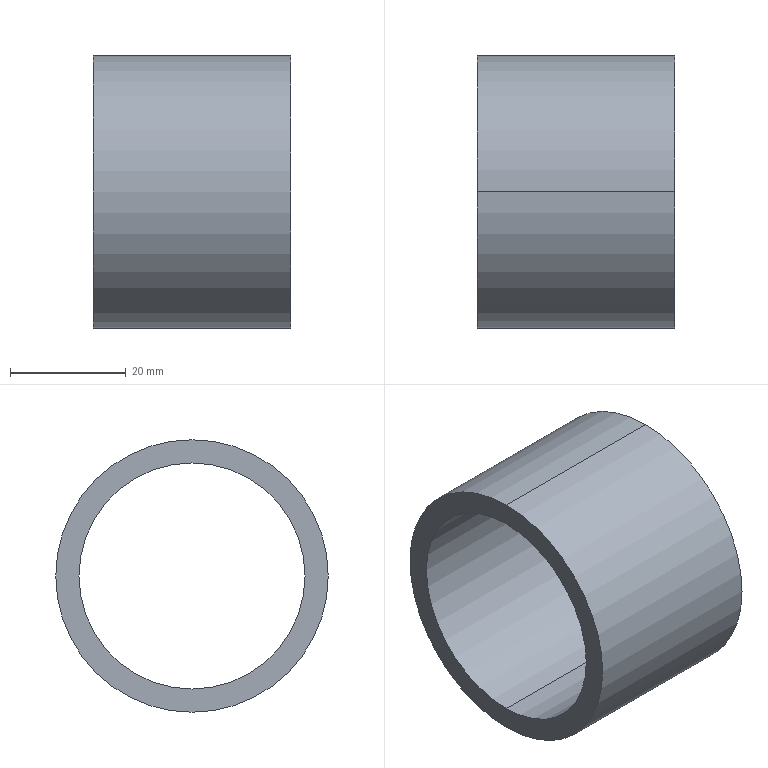Component | SolidWorks | 4-12-12ClampingAxisAssembly-1_4-12-6ClampingAxisBearingOuterPad-1 | 1 solid | 6 faces | box 34 x 47 x 47 mm | volume 18372 mm3 | cylinder 4 | plane 2 | commonest cylinder face diameters 39 x2 47 x2
build123d program:
from build123d import *

# Parameters (mm, degrees)
SKETCH1_R      = 23.5
SKETCH1_R_2    = 19.5
EXTRUDE1_DEPTH = 34


with BuildPart() as part:
    # Sketch1 → Extrude1 (new body)
    with BuildSketch(Plane(origin=(0, 0, 0), x_dir=(1, 0, 0), z_dir=(0, 1, 0))):
        with Locations(Location((0, 0, 0), (0, 0, 270))):
            Circle(SKETCH1_R)
        with Locations(Location((0, 0, 0), (0, 0, 270))):
            Circle(SKETCH1_R_2, mode=Mode.SUBTRACT)
    extrude(amount=EXTRUDE1_DEPTH)


solid = part.part

# Placed as in the assembly
solid = solid.moved(Location((-67.809, -4.181, 0), (0, 0, 90)))
STEP:
#1=COLOUR_RGB('',0.7922,0.8196,0.9333);
#2=FILL_AREA_STYLE_COLOUR('',#1);
#3=FILL_AREA_STYLE('',(#2));
#4=SURFACE_STYLE_FILL_AREA(#3);
#5=SURFACE_SIDE_STYLE('',(#4));
#6=SURFACE_STYLE_USAGE(.BOTH.,#5);
#7=PRESENTATION_STYLE_ASSIGNMENT((#6));
#8=CARTESIAN_POINT('',(-4.008,-0.1646,-0.7677));
#9=VERTEX_POINT('',#8);
#10=CARTESIAN_POINT('',(-4.008,-0.1646,0.7677));
#11=VERTEX_POINT('',#10);
#12=CARTESIAN_POINT('',(-4.008,-0.1646,0.));
#13=DIRECTION('',(-1.,-0.,-0.));
#14=DIRECTION('',(0.,0.,1.));
#15=AXIS2_PLACEMENT_3D('',#12,#13,#14);
#16=CIRCLE('',#15,0.7677);
#17=EDGE_CURVE('',#9,#11,#16,.T.);
#18=ORIENTED_EDGE('',*,*,#17,.T.);
#19=CARTESIAN_POINT('',(-2.67,-0.1646,0.7677));
#20=VERTEX_POINT('',#19);
#21=CARTESIAN_POINT('',(-4.008,-0.1646,0.7677));
#22=DIRECTION('',(1.,0.,0.));
#23=VECTOR('',#22,39.37);
#24=LINE('',#21,#23);
#25=EDGE_CURVE('',#11,#20,#24,.T.);
#26=ORIENTED_EDGE('',*,*,#25,.T.);
#27=CARTESIAN_POINT('',(-2.67,-0.1646,-0.7677));
#28=VERTEX_POINT('',#27);
#29=CARTESIAN_POINT('',(-2.67,-0.1646,0.));
#30=DIRECTION('',(-1.,-0.,-0.));
#31=DIRECTION('',(0.,0.,1.));
#32=AXIS2_PLACEMENT_3D('',#29,#30,#31);
#33=CIRCLE('',#32,0.7677);
#34=EDGE_CURVE('',#28,#20,#33,.T.);
#35=ORIENTED_EDGE('',*,*,#34,.F.);
#36=CARTESIAN_POINT('',(-4.008,-0.1646,-0.7677));
#37=DIRECTION('',(1.,0.,0.));
#38=VECTOR('',#37,39.37);
#39=LINE('',#36,#38);
#40=EDGE_CURVE('',#9,#28,#39,.T.);
#41=ORIENTED_EDGE('',*,*,#40,.F.);
#42=EDGE_LOOP('',(#18,#26,#35,#41));
#43=FACE_OUTER_BOUND('',#42,.T.);
#44=CARTESIAN_POINT('',(-4.008,-0.1646,0.));
#45=DIRECTION('',(1.,0.,0.));
#46=DIRECTION('',(0.,-0.,-1.));
#47=AXIS2_PLACEMENT_3D('',#44,#45,#46);
#48=CYLINDRICAL_SURFACE('',#47,0.7677);
#49=ADVANCED_FACE('',(#43),#48,.F.);
#50=CARTESIAN_POINT('',(-4.008,-0.1646,0.9252));
#51=VERTEX_POINT('',#50);
#52=CARTESIAN_POINT('',(-4.008,-0.1646,-0.9252));
#53=VERTEX_POINT('',#52);
#54=CARTESIAN_POINT('',(-4.008,-0.1646,0.));
#55=DIRECTION('',(-1.,-0.,-0.));
#56=DIRECTION('',(0.,0.,1.));
#57=AXIS2_PLACEMENT_3D('',#54,#55,#56);
#58=CIRCLE('',#57,0.9252);
#59=EDGE_CURVE('',#51,#53,#58,.T.);
#60=ORIENTED_EDGE('',*,*,#59,.F.);
#61=CARTESIAN_POINT('',(-2.67,-0.1646,0.9252));
#62=VERTEX_POINT('',#61);
#63=CARTESIAN_POINT('',(-4.008,-0.1646,0.9252));
#64=DIRECTION('',(1.,0.,0.));
#65=VECTOR('',#64,39.37);
#66=LINE('',#63,#65);
#67=EDGE_CURVE('',#51,#62,#66,.T.);
#68=ORIENTED_EDGE('',*,*,#67,.T.);
#69=CARTESIAN_POINT('',(-2.67,-0.1646,-0.9252));
#70=VERTEX_POINT('',#69);
#71=CARTESIAN_POINT('',(-2.67,-0.1646,0.));
#72=DIRECTION('',(-1.,-0.,-0.));
#73=DIRECTION('',(0.,0.,1.));
#74=AXIS2_PLACEMENT_3D('',#71,#72,#73);
#75=CIRCLE('',#74,0.9252);
#76=EDGE_CURVE('',#62,#70,#75,.T.);
#77=ORIENTED_EDGE('',*,*,#76,.T.);
#78=CARTESIAN_POINT('',(-4.008,-0.1646,-0.9252));
#79=DIRECTION('',(1.,0.,0.));
#80=VECTOR('',#79,39.37);
#81=LINE('',#78,#80);
#82=EDGE_CURVE('',#53,#70,#81,.T.);
#83=ORIENTED_EDGE('',*,*,#82,.F.);
#84=EDGE_LOOP('',(#60,#68,#77,#83));
#85=FACE_OUTER_BOUND('',#84,.T.);
#86=CARTESIAN_POINT('',(-4.008,-0.1646,0.));
#87=DIRECTION('',(1.,0.,0.));
#88=DIRECTION('',(0.,-0.,-1.));
#89=AXIS2_PLACEMENT_3D('',#86,#87,#88);
#90=CYLINDRICAL_SURFACE('',#89,0.9252);
#91=ADVANCED_FACE('',(#85),#90,.T.);
#92=CARTESIAN_POINT('',(-4.008,-0.1646,0.));
#93=DIRECTION('',(-1.,-0.,-0.));
#94=DIRECTION('',(0.,0.,1.));
#95=AXIS2_PLACEMENT_3D('',#92,#93,#94);
#96=CIRCLE('',#95,0.9252);
#97=EDGE_CURVE('',#53,#51,#96,.T.);
#98=ORIENTED_EDGE('',*,*,#97,.T.);
#99=ORIENTED_EDGE('',*,*,#59,.T.);
#100=EDGE_LOOP('',(#98,#99));
#101=FACE_OUTER_BOUND('',#100,.T.);
#102=ORIENTED_EDGE('',*,*,#17,.F.);
#103=CARTESIAN_POINT('',(-4.008,-0.1646,0.));
#104=DIRECTION('',(-1.,-0.,-0.));
#105=DIRECTION('',(0.,0.,1.));
#106=AXIS2_PLACEMENT_3D('',#103,#104,#105);
#107=CIRCLE('',#106,0.7677);
#108=EDGE_CURVE('',#11,#9,#107,.T.);
#109=ORIENTED_EDGE('',*,*,#108,.F.);
#110=EDGE_LOOP('',(#102,#109));
#111=FACE_BOUND('',#110,.T.);
#112=CARTESIAN_POINT('',(-4.008,-0.1646,0.));
#113=DIRECTION('',(-1.,-0.,-0.));
#114=DIRECTION('',(-0.,0.,1.));
#115=AXIS2_PLACEMENT_3D('',#112,#113,#114);
#116=PLANE('',#115);
#117=ADVANCED_FACE('',(#101,#111),#116,.T.);
#118=CARTESIAN_POINT('',(-2.67,-0.1646,0.));
#119=DIRECTION('',(-1.,-0.,-0.));
#120=DIRECTION('',(0.,0.,1.));
#121=AXIS2_PLACEMENT_3D('',#118,#119,#120);
#122=CIRCLE('',#121,0.9252);
#123=EDGE_CURVE('',#70,#62,#122,.T.);
#124=ORIENTED_EDGE('',*,*,#123,.F.);
#125=ORIENTED_EDGE('',*,*,#76,.F.);
#126=EDGE_LOOP('',(#124,#125));
#127=FACE_OUTER_BOUND('',#126,.T.);
#128=ORIENTED_EDGE('',*,*,#34,.T.);
#129=CARTESIAN_POINT('',(-2.67,-0.1646,0.));
#130=DIRECTION('',(-1.,-0.,-0.));
#131=DIRECTION('',(0.,0.,1.));
#132=AXIS2_PLACEMENT_3D('',#129,#130,#131);
#133=CIRCLE('',#132,0.7677);
#134=EDGE_CURVE('',#20,#28,#133,.T.);
#135=ORIENTED_EDGE('',*,*,#134,.T.);
#136=EDGE_LOOP('',(#128,#135));
#137=FACE_BOUND('',#136,.T.);
#138=CARTESIAN_POINT('',(-2.67,-0.1646,0.));
#139=DIRECTION('',(-1.,-0.,-0.));
#140=DIRECTION('',(-0.,0.,1.));
#141=AXIS2_PLACEMENT_3D('',#138,#139,#140);
#142=PLANE('',#141);
#143=ADVANCED_FACE('',(#127,#137),#142,.F.);
#144=ORIENTED_EDGE('',*,*,#67,.F.);
#145=ORIENTED_EDGE('',*,*,#97,.F.);
#146=ORIENTED_EDGE('',*,*,#82,.T.);
#147=ORIENTED_EDGE('',*,*,#123,.T.);
#148=EDGE_LOOP('',(#144,#145,#146,#147));
#149=FACE_OUTER_BOUND('',#148,.T.);
#150=CARTESIAN_POINT('',(-4.008,-0.1646,0.));
#151=DIRECTION('',(1.,0.,0.));
#152=DIRECTION('',(0.,-0.,-1.));
#153=AXIS2_PLACEMENT_3D('',#150,#151,#152);
#154=CYLINDRICAL_SURFACE('',#153,0.9252);
#155=ADVANCED_FACE('',(#149),#154,.T.);
#156=ORIENTED_EDGE('',*,*,#25,.F.);
#157=ORIENTED_EDGE('',*,*,#108,.T.);
#158=ORIENTED_EDGE('',*,*,#40,.T.);
#159=ORIENTED_EDGE('',*,*,#134,.F.);
#160=EDGE_LOOP('',(#156,#157,#158,#159));
#161=FACE_OUTER_BOUND('',#160,.T.);
#162=CARTESIAN_POINT('',(-4.008,-0.1646,0.));
#163=DIRECTION('',(1.,0.,0.));
#164=DIRECTION('',(0.,-0.,-1.));
#165=AXIS2_PLACEMENT_3D('',#162,#163,#164);
#166=CYLINDRICAL_SURFACE('',#165,0.7677);
#167=ADVANCED_FACE('',(#161),#166,.F.);
#168=CLOSED_SHELL('',(#49,#91,#117,#143,#155,#167));
#169=MANIFOLD_SOLID_BREP('',#168);
#170=STYLED_ITEM('',(#7),#169);
#171=(LENGTH_UNIT()NAMED_UNIT(*)SI_UNIT($,.METRE.));
#172=LENGTH_MEASURE_WITH_UNIT(LENGTH_MEASURE(0.0254),#171);
#173=DIMENSIONAL_EXPONENTS(1.,0.,0.,0.,0.,0.,0.);
#174=(CONVERSION_BASED_UNIT('',#172)LENGTH_UNIT()NAMED_UNIT(#173));
#175=UNCERTAINTY_MEASURE_WITH_UNIT(LENGTH_MEASURE(0.00001),#174,'','');
#176=(NAMED_UNIT(*)PLANE_ANGLE_UNIT()SI_UNIT($,.RADIAN.));
#177=(NAMED_UNIT(*)SI_UNIT($,.STERADIAN.)SOLID_ANGLE_UNIT());
#178=(GEOMETRIC_REPRESENTATION_CONTEXT(3)GLOBAL_UNCERTAINTY_ASSIGNED_CONTEXT((#175))GLOBAL_UNIT_ASSIGNED_CONTEXT((#174,#176,#177))REPRESENTATION_CONTEXT('',''));
#179=MECHANICAL_DESIGN_GEOMETRIC_PRESENTATION_REPRESENTATION('',(#170),#178);
#180=PRESENTATION_LAYER_ASSIGNMENT('','',(#170));
#181=CARTESIAN_POINT('',(0.,0.,0.));
#182=DIRECTION('',(0.,0.,1.));
#183=DIRECTION('',(1.,0.,0.));
#184=AXIS2_PLACEMENT_3D('',#181,#182,#183);
#185=(LENGTH_UNIT()NAMED_UNIT(*)SI_UNIT($,.METRE.));
#186=LENGTH_MEASURE_WITH_UNIT(LENGTH_MEASURE(0.0254),#185);
#187=DIMENSIONAL_EXPONENTS(1.,0.,0.,0.,0.,0.,0.);
#188=(CONVERSION_BASED_UNIT('',#186)LENGTH_UNIT()NAMED_UNIT(#187));
#189=UNCERTAINTY_MEASURE_WITH_UNIT(LENGTH_MEASURE(0.00001),#188,'','');
#190=(NAMED_UNIT(*)PLANE_ANGLE_UNIT()SI_UNIT($,.RADIAN.));
#191=(NAMED_UNIT(*)SI_UNIT($,.STERADIAN.)SOLID_ANGLE_UNIT());
#192=(GEOMETRIC_REPRESENTATION_CONTEXT(3)GLOBAL_UNCERTAINTY_ASSIGNED_CONTEXT((#189))GLOBAL_UNIT_ASSIGNED_CONTEXT((#188,#190,#191))REPRESENTATION_CONTEXT('',''));
#193=ADVANCED_BREP_SHAPE_REPRESENTATION('',(#169,#184),#192);